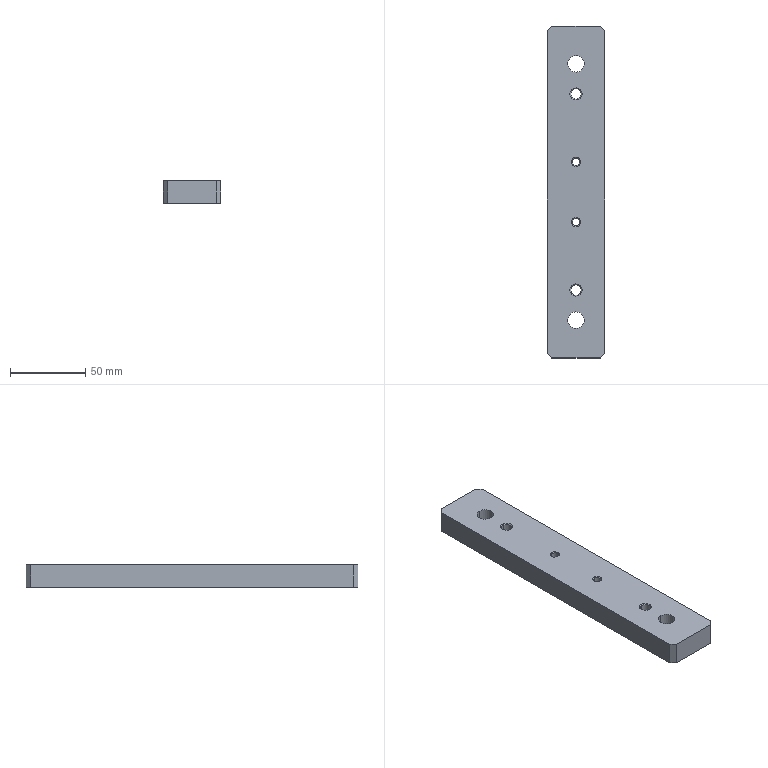Component | SolidWorks | TransitionPlate-1 | 1 solid | 30 faces | box 38 x 220 x 15 mm | volume 120587 mm3 | cylinder 12 | plane 10 | cone 8 | commonest cylinder face diameters 5 x4 6.8 x4 11 x4
build123d program:
from build123d import *

# Parameters (mm, degrees)
BOSS_EXTRUDE1_DEPTH                                  = 15
F_11_0_11_DIAMETER_HOLE1_D                           = 11
CONICAL_COUNTERSUNK_HOLE_1_FOR_M6_FLAT_H_D           = 6.8
CONICAL_COUNTERSUNK_HOLE_1_FOR_M6_FLAT_H_CSINK_D     = 8.05
CONICAL_COUNTERSUNK_HOLE_1_FOR_M6_FLAT_H_CSINK_ANGLE = 90
F_5_0_5_DIAMETER_HOLE1_D                             = 5
F_5_0_5_DIAMETER_HOLE1_CSINK_D                       = 6.05
F_5_0_5_DIAMETER_HOLE1_CSINK_ANGLE                   = 90


with BuildPart() as part:
    # Sketch1 → Boss-Extrude1 (new body)
    with BuildSketch(Plane.XY.offset(7.5)):
        Polygon((-110, 16), (-110, -16), (-107, -19), (107, -19), (110, -16), (110, 16), (107, 19), (-107, 19), align=None)
    extrude(amount=-BOSS_EXTRUDE1_DEPTH)

    # 11.0 _11_ Diameter Hole1 (through all)
    with Locations(Plane(origin=(0, 0, -7.5), x_dir=(-1, 0, 0), z_dir=(0, 0, -1))):
        with Locations((-85, 0), (85, 0)):
            Hole(F_11_0_11_DIAMETER_HOLE1_D / 2)

    # Conical Countersunk Hole 1 for M6 Flat H (through all)
    with Locations(Plane.XY.offset(7.5)):
        with Locations((65, 0), (-65, 0)):
            CounterSinkHole(CONICAL_COUNTERSUNK_HOLE_1_FOR_M6_FLAT_H_D / 2, CONICAL_COUNTERSUNK_HOLE_1_FOR_M6_FLAT_H_CSINK_D / 2, counter_sink_angle=CONICAL_COUNTERSUNK_HOLE_1_FOR_M6_FLAT_H_CSINK_ANGLE)

    # 5.0 _5_ Diameter Hole1 (through all)
    with Locations(Plane.XY.offset(7.5)):
        with Locations((20, 0), (-20, 0)):
            CounterSinkHole(F_5_0_5_DIAMETER_HOLE1_D / 2, F_5_0_5_DIAMETER_HOLE1_CSINK_D / 2, counter_sink_angle=F_5_0_5_DIAMETER_HOLE1_CSINK_ANGLE)


solid = part.part

# Placed as in the assembly
solid = solid.moved(Location((0, 0, 263.054), (0, 0, 90)))
STEP:
#1=COLOUR_RGB('',0.7922,0.8196,0.9333);
#2=FILL_AREA_STYLE_COLOUR('',#1);
#3=FILL_AREA_STYLE('',(#2));
#4=SURFACE_STYLE_FILL_AREA(#3);
#5=SURFACE_SIDE_STYLE('',(#4));
#6=SURFACE_STYLE_USAGE(.BOTH.,#5);
#7=PRESENTATION_STYLE_ASSIGNMENT((#6));
#8=CARTESIAN_POINT('',(-0.,-0.689,10.631));
#9=VERTEX_POINT('',#8);
#10=CARTESIAN_POINT('',(-0.,-0.8858,10.631));
#11=VERTEX_POINT('',#10);
#12=CARTESIAN_POINT('',(-0.,-0.7874,10.631));
#13=DIRECTION('',(-0.,0.,1.));
#14=DIRECTION('',(-0.,-1.,0.));
#15=AXIS2_PLACEMENT_3D('',#12,#13,#14);
#16=CIRCLE('',#15,0.09843);
#17=EDGE_CURVE('',#9,#11,#16,.T.);
#18=ORIENTED_EDGE('',*,*,#17,.F.);
#19=CARTESIAN_POINT('',(-0.,-0.6683,10.652));
#20=VERTEX_POINT('',#19);
#21=CARTESIAN_POINT('',(-0.,-0.6683,10.652));
#22=DIRECTION('',(0.,0.7071,0.7071));
#23=VECTOR('',#22,39.37);
#24=LINE('',#21,#23);
#25=EDGE_CURVE('',#9,#20,#24,.T.);
#26=ORIENTED_EDGE('',*,*,#25,.T.);
#27=CARTESIAN_POINT('',(-0.,-0.9065,10.652));
#28=VERTEX_POINT('',#27);
#29=CARTESIAN_POINT('',(-0.,-0.7874,10.652));
#30=DIRECTION('',(-0.,0.,1.));
#31=DIRECTION('',(-0.,-1.,0.));
#32=AXIS2_PLACEMENT_3D('',#29,#30,#31);
#33=CIRCLE('',#32,0.1191);
#34=EDGE_CURVE('',#20,#28,#33,.T.);
#35=ORIENTED_EDGE('',*,*,#34,.T.);
#36=CARTESIAN_POINT('',(-0.,-0.9065,10.652));
#37=DIRECTION('',(-0.,-0.7071,0.7071));
#38=VECTOR('',#37,39.37);
#39=LINE('',#36,#38);
#40=EDGE_CURVE('',#11,#28,#39,.T.);
#41=ORIENTED_EDGE('',*,*,#40,.F.);
#42=EDGE_LOOP('',(#18,#26,#35,#41));
#43=FACE_OUTER_BOUND('',#42,.T.);
#44=CARTESIAN_POINT('',(-0.,-0.7874,10.652));
#45=DIRECTION('',(-0.,0.,1.));
#46=DIRECTION('',(-0.,-1.,0.));
#47=AXIS2_PLACEMENT_3D('',#44,#45,#46);
#48=CONICAL_SURFACE('',#47,0.1191,0.7854);
#49=ADVANCED_FACE('',(#43),#48,.F.);
#50=CARTESIAN_POINT('',(-0.,-0.689,10.061));
#51=VERTEX_POINT('',#50);
#52=CARTESIAN_POINT('',(-0.,-0.8858,10.061));
#53=VERTEX_POINT('',#52);
#54=CARTESIAN_POINT('',(-0.,-0.7874,10.061));
#55=DIRECTION('',(-0.,0.,1.));
#56=DIRECTION('',(-0.,-1.,0.));
#57=AXIS2_PLACEMENT_3D('',#54,#55,#56);
#58=CIRCLE('',#57,0.09843);
#59=EDGE_CURVE('',#51,#53,#58,.T.);
#60=ORIENTED_EDGE('',*,*,#59,.F.);
#61=CARTESIAN_POINT('',(-0.,-0.689,10.652));
#62=DIRECTION('',(-0.,0.,1.));
#63=VECTOR('',#62,39.37);
#64=LINE('',#61,#63);
#65=EDGE_CURVE('',#51,#9,#64,.T.);
#66=ORIENTED_EDGE('',*,*,#65,.T.);
#67=ORIENTED_EDGE('',*,*,#17,.T.);
#68=CARTESIAN_POINT('',(-0.,-0.8858,10.652));
#69=DIRECTION('',(-0.,0.,1.));
#70=VECTOR('',#69,39.37);
#71=LINE('',#68,#70);
#72=EDGE_CURVE('',#53,#11,#71,.T.);
#73=ORIENTED_EDGE('',*,*,#72,.F.);
#74=EDGE_LOOP('',(#60,#66,#67,#73));
#75=FACE_OUTER_BOUND('',#74,.T.);
#76=CARTESIAN_POINT('',(-0.,-0.7874,10.652));
#77=DIRECTION('',(-0.,0.,1.));
#78=DIRECTION('',(-0.,-1.,0.));
#79=AXIS2_PLACEMENT_3D('',#76,#77,#78);
#80=CYLINDRICAL_SURFACE('',#79,0.09843);
#81=ADVANCED_FACE('',(#75),#80,.F.);
#82=CARTESIAN_POINT('',(-0.,0.8858,10.631));
#83=VERTEX_POINT('',#82);
#84=CARTESIAN_POINT('',(-0.,0.689,10.631));
#85=VERTEX_POINT('',#84);
#86=CARTESIAN_POINT('',(-0.,0.7874,10.631));
#87=DIRECTION('',(-0.,0.,1.));
#88=DIRECTION('',(-0.,-1.,0.));
#89=AXIS2_PLACEMENT_3D('',#86,#87,#88);
#90=CIRCLE('',#89,0.09843);
#91=EDGE_CURVE('',#83,#85,#90,.T.);
#92=ORIENTED_EDGE('',*,*,#91,.F.);
#93=CARTESIAN_POINT('',(-0.,0.9065,10.652));
#94=VERTEX_POINT('',#93);
#95=CARTESIAN_POINT('',(-0.,0.9065,10.652));
#96=DIRECTION('',(0.,0.7071,0.7071));
#97=VECTOR('',#96,39.37);
#98=LINE('',#95,#97);
#99=EDGE_CURVE('',#83,#94,#98,.T.);
#100=ORIENTED_EDGE('',*,*,#99,.T.);
#101=CARTESIAN_POINT('',(-0.,0.6683,10.652));
#102=VERTEX_POINT('',#101);
#103=CARTESIAN_POINT('',(-0.,0.7874,10.652));
#104=DIRECTION('',(-0.,0.,1.));
#105=DIRECTION('',(-0.,-1.,0.));
#106=AXIS2_PLACEMENT_3D('',#103,#104,#105);
#107=CIRCLE('',#106,0.1191);
#108=EDGE_CURVE('',#94,#102,#107,.T.);
#109=ORIENTED_EDGE('',*,*,#108,.T.);
#110=CARTESIAN_POINT('',(-0.,0.6683,10.652));
#111=DIRECTION('',(-0.,-0.7071,0.7071));
#112=VECTOR('',#111,39.37);
#113=LINE('',#110,#112);
#114=EDGE_CURVE('',#85,#102,#113,.T.);
#115=ORIENTED_EDGE('',*,*,#114,.F.);
#116=EDGE_LOOP('',(#92,#100,#109,#115));
#117=FACE_OUTER_BOUND('',#116,.T.);
#118=CARTESIAN_POINT('',(-0.,0.7874,10.652));
#119=DIRECTION('',(-0.,0.,1.));
#120=DIRECTION('',(-0.,-1.,0.));
#121=AXIS2_PLACEMENT_3D('',#118,#119,#120);
#122=CONICAL_SURFACE('',#121,0.1191,0.7854);
#123=ADVANCED_FACE('',(#117),#122,.F.);
#124=CARTESIAN_POINT('',(-0.,0.8858,10.061));
#125=VERTEX_POINT('',#124);
#126=CARTESIAN_POINT('',(-0.,0.689,10.061));
#127=VERTEX_POINT('',#126);
#128=CARTESIAN_POINT('',(-0.,0.7874,10.061));
#129=DIRECTION('',(-0.,0.,1.));
#130=DIRECTION('',(-0.,-1.,0.));
#131=AXIS2_PLACEMENT_3D('',#128,#129,#130);
#132=CIRCLE('',#131,0.09843);
#133=EDGE_CURVE('',#125,#127,#132,.T.);
#134=ORIENTED_EDGE('',*,*,#133,.F.);
#135=CARTESIAN_POINT('',(-0.,0.8858,10.652));
#136=DIRECTION('',(-0.,0.,1.));
#137=VECTOR('',#136,39.37);
#138=LINE('',#135,#137);
#139=EDGE_CURVE('',#125,#83,#138,.T.);
#140=ORIENTED_EDGE('',*,*,#139,.T.);
#141=ORIENTED_EDGE('',*,*,#91,.T.);
#142=CARTESIAN_POINT('',(-0.,0.689,10.652));
#143=DIRECTION('',(-0.,0.,1.));
#144=VECTOR('',#143,39.37);
#145=LINE('',#142,#144);
#146=EDGE_CURVE('',#127,#85,#145,.T.);
#147=ORIENTED_EDGE('',*,*,#146,.F.);
#148=EDGE_LOOP('',(#134,#140,#141,#147));
#149=FACE_OUTER_BOUND('',#148,.T.);
#150=CARTESIAN_POINT('',(-0.,0.7874,10.652));
#151=DIRECTION('',(-0.,0.,1.));
#152=DIRECTION('',(-0.,-1.,0.));
#153=AXIS2_PLACEMENT_3D('',#150,#151,#152);
#154=CYLINDRICAL_SURFACE('',#153,0.09843);
#155=ADVANCED_FACE('',(#149),#154,.F.);
#156=CARTESIAN_POINT('',(-0.,-2.425,10.627));
#157=VERTEX_POINT('',#156);
#158=CARTESIAN_POINT('',(-0.,-2.693,10.627));
#159=VERTEX_POINT('',#158);
#160=CARTESIAN_POINT('',(-0.,-2.559,10.627));
#161=DIRECTION('',(-0.,0.,1.));
#162=DIRECTION('',(-0.,-1.,0.));
#163=AXIS2_PLACEMENT_3D('',#160,#161,#162);
#164=CIRCLE('',#163,0.1339);
#165=EDGE_CURVE('',#157,#159,#164,.T.);
#166=ORIENTED_EDGE('',*,*,#165,.F.);
#167=CARTESIAN_POINT('',(-0.,-2.401,10.652));
#168=VERTEX_POINT('',#167);
#169=CARTESIAN_POINT('',(-0.,-2.401,10.652));
#170=DIRECTION('',(0.,0.7071,0.7071));
#171=VECTOR('',#170,39.37);
#172=LINE('',#169,#171);
#173=EDGE_CURVE('',#157,#168,#172,.T.);
#174=ORIENTED_EDGE('',*,*,#173,.T.);
#175=CARTESIAN_POINT('',(-0.,-2.718,10.652));
#176=VERTEX_POINT('',#175);
#177=CARTESIAN_POINT('',(-0.,-2.559,10.652));
#178=DIRECTION('',(-0.,0.,1.));
#179=DIRECTION('',(-0.,-1.,0.));
#180=AXIS2_PLACEMENT_3D('',#177,#178,#179);
#181=CIRCLE('',#180,0.1585);
#182=EDGE_CURVE('',#168,#176,#181,.T.);
#183=ORIENTED_EDGE('',*,*,#182,.T.);
#184=CARTESIAN_POINT('',(-0.,-2.718,10.652));
#185=DIRECTION('',(-0.,-0.7071,0.7071));
#186=VECTOR('',#185,39.37);
#187=LINE('',#184,#186);
#188=EDGE_CURVE('',#159,#176,#187,.T.);
#189=ORIENTED_EDGE('',*,*,#188,.F.);
#190=EDGE_LOOP('',(#166,#174,#183,#189));
#191=FACE_OUTER_BOUND('',#190,.T.);
#192=CARTESIAN_POINT('',(-0.,-2.559,10.652));
#193=DIRECTION('',(-0.,0.,1.));
#194=DIRECTION('',(-0.,-1.,0.));
#195=AXIS2_PLACEMENT_3D('',#192,#193,#194);
#196=CONICAL_SURFACE('',#195,0.1585,0.7854);
#197=ADVANCED_FACE('',(#191),#196,.F.);
#198=CARTESIAN_POINT('',(-0.,-2.425,10.061));
#199=VERTEX_POINT('',#198);
#200=CARTESIAN_POINT('',(-0.,-2.693,10.061));
#201=VERTEX_POINT('',#200);
#202=CARTESIAN_POINT('',(-0.,-2.559,10.061));
#203=DIRECTION('',(-0.,0.,1.));
#204=DIRECTION('',(-0.,-1.,0.));
#205=AXIS2_PLACEMENT_3D('',#202,#203,#204);
#206=CIRCLE('',#205,0.1339);
#207=EDGE_CURVE('',#199,#201,#206,.T.);
#208=ORIENTED_EDGE('',*,*,#207,.F.);
#209=CARTESIAN_POINT('',(-0.,-2.425,10.652));
#210=DIRECTION('',(-0.,0.,1.));
#211=VECTOR('',#210,39.37);
#212=LINE('',#209,#211);
#213=EDGE_CURVE('',#199,#157,#212,.T.);
#214=ORIENTED_EDGE('',*,*,#213,.T.);
#215=ORIENTED_EDGE('',*,*,#165,.T.);
#216=CARTESIAN_POINT('',(-0.,-2.693,10.652));
#217=DIRECTION('',(-0.,0.,1.));
#218=VECTOR('',#217,39.37);
#219=LINE('',#216,#218);
#220=EDGE_CURVE('',#201,#159,#219,.T.);
#221=ORIENTED_EDGE('',*,*,#220,.F.);
#222=EDGE_LOOP('',(#208,#214,#215,#221));
#223=FACE_OUTER_BOUND('',#222,.T.);
#224=CARTESIAN_POINT('',(-0.,-2.559,10.652));
#225=DIRECTION('',(-0.,0.,1.));
#226=DIRECTION('',(-0.,-1.,0.));
#227=AXIS2_PLACEMENT_3D('',#224,#225,#226);
#228=CYLINDRICAL_SURFACE('',#227,0.1339);
#229=ADVANCED_FACE('',(#223),#228,.F.);
#230=CARTESIAN_POINT('',(-0.,2.693,10.627));
#231=VERTEX_POINT('',#230);
#232=CARTESIAN_POINT('',(-0.,2.425,10.627));
#233=VERTEX_POINT('',#232);
#234=CARTESIAN_POINT('',(-0.,2.559,10.627));
#235=DIRECTION('',(-0.,0.,1.));
#236=DIRECTION('',(-0.,-1.,0.));
#237=AXIS2_PLACEMENT_3D('',#234,#235,#236);
#238=CIRCLE('',#237,0.1339);
#239=EDGE_CURVE('',#231,#233,#238,.T.);
#240=ORIENTED_EDGE('',*,*,#239,.F.);
#241=CARTESIAN_POINT('',(-0.,2.718,10.652));
#242=VERTEX_POINT('',#241);
#243=CARTESIAN_POINT('',(-0.,2.718,10.652));
#244=DIRECTION('',(0.,0.7071,0.7071));
#245=VECTOR('',#244,39.37);
#246=LINE('',#243,#245);
#247=EDGE_CURVE('',#231,#242,#246,.T.);
#248=ORIENTED_EDGE('',*,*,#247,.T.);
#249=CARTESIAN_POINT('',(-0.,2.401,10.652));
#250=VERTEX_POINT('',#249);
#251=CARTESIAN_POINT('',(-0.,2.559,10.652));
#252=DIRECTION('',(-0.,0.,1.));
#253=DIRECTION('',(-0.,-1.,0.));
#254=AXIS2_PLACEMENT_3D('',#251,#252,#253);
#255=CIRCLE('',#254,0.1585);
#256=EDGE_CURVE('',#242,#250,#255,.T.);
#257=ORIENTED_EDGE('',*,*,#256,.T.);
#258=CARTESIAN_POINT('',(-0.,2.401,10.652));
#259=DIRECTION('',(-0.,-0.7071,0.7071));
#260=VECTOR('',#259,39.37);
#261=LINE('',#258,#260);
#262=EDGE_CURVE('',#233,#250,#261,.T.);
#263=ORIENTED_EDGE('',*,*,#262,.F.);
#264=EDGE_LOOP('',(#240,#248,#257,#263));
#265=FACE_OUTER_BOUND('',#264,.T.);
#266=CARTESIAN_POINT('',(-0.,2.559,10.652));
#267=DIRECTION('',(-0.,0.,1.));
#268=DIRECTION('',(-0.,-1.,0.));
#269=AXIS2_PLACEMENT_3D('',#266,#267,#268);
#270=CONICAL_SURFACE('',#269,0.1585,0.7854);
#271=ADVANCED_FACE('',(#265),#270,.F.);
#272=CARTESIAN_POINT('',(-0.,2.693,10.061));
#273=VERTEX_POINT('',#272);
#274=CARTESIAN_POINT('',(-0.,2.425,10.061));
#275=VERTEX_POINT('',#274);
#276=CARTESIAN_POINT('',(-0.,2.559,10.061));
#277=DIRECTION('',(-0.,0.,1.));
#278=DIRECTION('',(-0.,-1.,0.));
#279=AXIS2_PLACEMENT_3D('',#276,#277,#278);
#280=CIRCLE('',#279,0.1339);
#281=EDGE_CURVE('',#273,#275,#280,.T.);
#282=ORIENTED_EDGE('',*,*,#281,.F.);
#283=CARTESIAN_POINT('',(-0.,2.693,10.652));
#284=DIRECTION('',(-0.,0.,1.));
#285=VECTOR('',#284,39.37);
#286=LINE('',#283,#285);
#287=EDGE_CURVE('',#273,#231,#286,.T.);
#288=ORIENTED_EDGE('',*,*,#287,.T.);
#289=ORIENTED_EDGE('',*,*,#239,.T.);
#290=CARTESIAN_POINT('',(-0.,2.425,10.652));
#291=DIRECTION('',(-0.,0.,1.));
#292=VECTOR('',#291,39.37);
#293=LINE('',#290,#292);
#294=EDGE_CURVE('',#275,#233,#293,.T.);
#295=ORIENTED_EDGE('',*,*,#294,.F.);
#296=EDGE_LOOP('',(#282,#288,#289,#295));
#297=FACE_OUTER_BOUND('',#296,.T.);
#298=CARTESIAN_POINT('',(-0.,2.559,10.652));
#299=DIRECTION('',(-0.,0.,1.));
#300=DIRECTION('',(-0.,-1.,0.));
#301=AXIS2_PLACEMENT_3D('',#298,#299,#300);
#302=CYLINDRICAL_SURFACE('',#301,0.1339);
#303=ADVANCED_FACE('',(#297),#302,.F.);
#304=CARTESIAN_POINT('',(-0.,-3.563,10.652));
#305=VERTEX_POINT('',#304);
#306=CARTESIAN_POINT('',(-0.,-3.13,10.652));
#307=VERTEX_POINT('',#306);
#308=CARTESIAN_POINT('',(-0.,-3.346,10.652));
#309=DIRECTION('',(0.,-0.,-1.));
#310=DIRECTION('',(0.,1.,0.));
#311=AXIS2_PLACEMENT_3D('',#308,#309,#310);
#312=CIRCLE('',#311,0.2165);
#313=EDGE_CURVE('',#305,#307,#312,.T.);
#314=ORIENTED_EDGE('',*,*,#313,.F.);
#315=CARTESIAN_POINT('',(-0.,-3.563,10.061));
#316=VERTEX_POINT('',#315);
#317=CARTESIAN_POINT('',(-0.,-3.563,10.061));
#318=DIRECTION('',(0.,-0.,-1.));
#319=VECTOR('',#318,39.37);
#320=LINE('',#317,#319);
#321=EDGE_CURVE('',#305,#316,#320,.T.);
#322=ORIENTED_EDGE('',*,*,#321,.T.);
#323=CARTESIAN_POINT('',(-0.,-3.13,10.061));
#324=VERTEX_POINT('',#323);
#325=CARTESIAN_POINT('',(-0.,-3.346,10.061));
#326=DIRECTION('',(0.,-0.,-1.));
#327=DIRECTION('',(0.,1.,0.));
#328=AXIS2_PLACEMENT_3D('',#325,#326,#327);
#329=CIRCLE('',#328,0.2165);
#330=EDGE_CURVE('',#316,#324,#329,.T.);
#331=ORIENTED_EDGE('',*,*,#330,.T.);
#332=CARTESIAN_POINT('',(-0.,-3.13,10.061));
#333=DIRECTION('',(0.,-0.,-1.));
#334=VECTOR('',#333,39.37);
#335=LINE('',#332,#334);
#336=EDGE_CURVE('',#307,#324,#335,.T.);
#337=ORIENTED_EDGE('',*,*,#336,.F.);
#338=EDGE_LOOP('',(#314,#322,#331,#337));
#339=FACE_OUTER_BOUND('',#338,.T.);
#340=CARTESIAN_POINT('',(-0.,-3.346,10.061));
#341=DIRECTION('',(0.,-0.,-1.));
#342=DIRECTION('',(0.,1.,0.));
#343=AXIS2_PLACEMENT_3D('',#340,#341,#342);
#344=CYLINDRICAL_SURFACE('',#343,0.2165);
#345=ADVANCED_FACE('',(#339),#344,.F.);
#346=CARTESIAN_POINT('',(-0.,3.13,10.652));
#347=VERTEX_POINT('',#346);
#348=CARTESIAN_POINT('',(-0.,3.563,10.652));
#349=VERTEX_POINT('',#348);
#350=CARTESIAN_POINT('',(-0.,3.346,10.652));
#351=DIRECTION('',(0.,-0.,-1.));
#352=DIRECTION('',(0.,1.,0.));
#353=AXIS2_PLACEMENT_3D('',#350,#351,#352);
#354=CIRCLE('',#353,0.2165);
#355=EDGE_CURVE('',#347,#349,#354,.T.);
#356=ORIENTED_EDGE('',*,*,#355,.F.);
#357=CARTESIAN_POINT('',(-0.,3.13,10.061));
#358=VERTEX_POINT('',#357);
#359=CARTESIAN_POINT('',(-0.,3.13,10.061));
#360=DIRECTION('',(0.,-0.,-1.));
#361=VECTOR('',#360,39.37);
#362=LINE('',#359,#361);
#363=EDGE_CURVE('',#347,#358,#362,.T.);
#364=ORIENTED_EDGE('',*,*,#363,.T.);
#365=CARTESIAN_POINT('',(-0.,3.563,10.061));
#366=VERTEX_POINT('',#365);
#367=CARTESIAN_POINT('',(-0.,3.346,10.061));
#368=DIRECTION('',(0.,-0.,-1.));
#369=DIRECTION('',(0.,1.,0.));
#370=AXIS2_PLACEMENT_3D('',#367,#368,#369);
#371=CIRCLE('',#370,0.2165);
#372=EDGE_CURVE('',#358,#366,#371,.T.);
#373=ORIENTED_EDGE('',*,*,#372,.T.);
#374=CARTESIAN_POINT('',(-0.,3.563,10.061));
#375=DIRECTION('',(0.,-0.,-1.));
#376=VECTOR('',#375,39.37);
#377=LINE('',#374,#376);
#378=EDGE_CURVE('',#349,#366,#377,.T.);
#379=ORIENTED_EDGE('',*,*,#378,.F.);
#380=EDGE_LOOP('',(#356,#364,#373,#379));
#381=FACE_OUTER_BOUND('',#380,.T.);
#382=CARTESIAN_POINT('',(-0.,3.346,10.061));
#383=DIRECTION('',(0.,-0.,-1.));
#384=DIRECTION('',(0.,1.,0.));
#385=AXIS2_PLACEMENT_3D('',#382,#383,#384);
#386=CYLINDRICAL_SURFACE('',#385,0.2165);
#387=ADVANCED_FACE('',(#381),#386,.F.);
#388=CARTESIAN_POINT('',(0.748,4.213,10.652));
#389=VERTEX_POINT('',#388);
#390=CARTESIAN_POINT('',(0.6299,4.331,10.652));
#391=VERTEX_POINT('',#390);
#392=CARTESIAN_POINT('',(0.748,4.213,10.652));
#393=DIRECTION('',(-0.7071,0.7071,-0.));
#394=VECTOR('',#393,39.37);
#395=LINE('',#392,#394);
#396=EDGE_CURVE('',#389,#391,#395,.T.);
#397=ORIENTED_EDGE('',*,*,#396,.F.);
#398=CARTESIAN_POINT('',(0.748,4.213,10.061));
#399=VERTEX_POINT('',#398);
#400=CARTESIAN_POINT('',(0.748,4.213,10.061));
#401=DIRECTION('',(-0.,0.,1.));
#402=VECTOR('',#401,39.37);
#403=LINE('',#400,#402);
#404=EDGE_CURVE('',#399,#389,#403,.T.);
#405=ORIENTED_EDGE('',*,*,#404,.F.);
#406=CARTESIAN_POINT('',(0.6299,4.331,10.061));
#407=VERTEX_POINT('',#406);
#408=CARTESIAN_POINT('',(0.748,4.213,10.061));
#409=DIRECTION('',(-0.7071,0.7071,-0.));
#410=VECTOR('',#409,39.37);
#411=LINE('',#408,#410);
#412=EDGE_CURVE('',#399,#407,#411,.T.);
#413=ORIENTED_EDGE('',*,*,#412,.T.);
#414=CARTESIAN_POINT('',(0.6299,4.331,10.061));
#415=DIRECTION('',(-0.,0.,1.));
#416=VECTOR('',#415,39.37);
#417=LINE('',#414,#416);
#418=EDGE_CURVE('',#407,#391,#417,.T.);
#419=ORIENTED_EDGE('',*,*,#418,.T.);
#420=EDGE_LOOP('',(#397,#405,#413,#419));
#421=FACE_OUTER_BOUND('',#420,.T.);
#422=CARTESIAN_POINT('',(0.748,4.213,10.061));
#423=DIRECTION('',(0.7071,0.7071,0.));
#424=DIRECTION('',(-0.7071,0.7071,-0.));
#425=AXIS2_PLACEMENT_3D('',#422,#423,#424);
#426=PLANE('',#425);
#427=ADVANCED_FACE('',(#421),#426,.T.);
#428=CARTESIAN_POINT('',(0.748,-4.213,10.652));
#429=VERTEX_POINT('',#428);
#430=CARTESIAN_POINT('',(0.748,-4.213,10.652));
#431=DIRECTION('',(0.,1.,-0.));
#432=VECTOR('',#431,39.37);
#433=LINE('',#430,#432);
#434=EDGE_CURVE('',#429,#389,#433,.T.);
#435=ORIENTED_EDGE('',*,*,#434,.F.);
#436=CARTESIAN_POINT('',(0.748,-4.213,10.061));
#437=VERTEX_POINT('',#436);
#438=CARTESIAN_POINT('',(0.748,-4.213,10.061));
#439=DIRECTION('',(-0.,0.,1.));
#440=VECTOR('',#439,39.37);
#441=LINE('',#438,#440);
#442=EDGE_CURVE('',#437,#429,#441,.T.);
#443=ORIENTED_EDGE('',*,*,#442,.F.);
#444=CARTESIAN_POINT('',(0.748,-4.213,10.061));
#445=DIRECTION('',(0.,1.,-0.));
#446=VECTOR('',#445,39.37);
#447=LINE('',#444,#446);
#448=EDGE_CURVE('',#437,#399,#447,.T.);
#449=ORIENTED_EDGE('',*,*,#448,.T.);
#450=ORIENTED_EDGE('',*,*,#404,.T.);
#451=EDGE_LOOP('',(#435,#443,#449,#450));
#452=FACE_OUTER_BOUND('',#451,.T.);
#453=CARTESIAN_POINT('',(0.748,-4.213,10.061));
#454=DIRECTION('',(1.,-0.,0.));
#455=DIRECTION('',(-0.,0.,1.));
#456=AXIS2_PLACEMENT_3D('',#453,#454,#455);
#457=PLANE('',#456);
#458=ADVANCED_FACE('',(#452),#457,.T.);
#459=CARTESIAN_POINT('',(0.6299,-4.331,10.652));
#460=VERTEX_POINT('',#459);
#461=CARTESIAN_POINT('',(0.6299,-4.331,10.652));
#462=DIRECTION('',(0.7071,0.7071,0.));
#463=VECTOR('',#462,39.37);
#464=LINE('',#461,#463);
#465=EDGE_CURVE('',#460,#429,#464,.T.);
#466=ORIENTED_EDGE('',*,*,#465,.F.);
#467=CARTESIAN_POINT('',(0.6299,-4.331,10.061));
#468=VERTEX_POINT('',#467);
#469=CARTESIAN_POINT('',(0.6299,-4.331,10.061));
#470=DIRECTION('',(-0.,0.,1.));
#471=VECTOR('',#470,39.37);
#472=LINE('',#469,#471);
#473=EDGE_CURVE('',#468,#460,#472,.T.);
#474=ORIENTED_EDGE('',*,*,#473,.F.);
#475=CARTESIAN_POINT('',(0.6299,-4.331,10.061));
#476=DIRECTION('',(0.7071,0.7071,0.));
#477=VECTOR('',#476,39.37);
#478=LINE('',#475,#477);
#479=EDGE_CURVE('',#468,#437,#478,.T.);
#480=ORIENTED_EDGE('',*,*,#479,.T.);
#481=ORIENTED_EDGE('',*,*,#442,.T.);
#482=EDGE_LOOP('',(#466,#474,#480,#481));
#483=FACE_OUTER_BOUND('',#482,.T.);
#484=CARTESIAN_POINT('',(0.6299,-4.331,10.061));
#485=DIRECTION('',(0.7071,-0.7071,0.));
#486=DIRECTION('',(0.7071,0.7071,0.));
#487=AXIS2_PLACEMENT_3D('',#484,#485,#486);
#488=PLANE('',#487);
#489=ADVANCED_FACE('',(#483),#488,.T.);
#490=CARTESIAN_POINT('',(-0.6299,-4.331,10.652));
#491=VERTEX_POINT('',#490);
#492=CARTESIAN_POINT('',(-0.6299,-4.331,10.652));
#493=DIRECTION('',(1.,-0.,0.));
#494=VECTOR('',#493,39.37);
#495=LINE('',#492,#494);
#496=EDGE_CURVE('',#491,#460,#495,.T.);
#497=ORIENTED_EDGE('',*,*,#496,.F.);
#498=CARTESIAN_POINT('',(-0.6299,-4.331,10.061));
#499=VERTEX_POINT('',#498);
#500=CARTESIAN_POINT('',(-0.6299,-4.331,10.061));
#501=DIRECTION('',(-0.,0.,1.));
#502=VECTOR('',#501,39.37);
#503=LINE('',#500,#502);
#504=EDGE_CURVE('',#499,#491,#503,.T.);
#505=ORIENTED_EDGE('',*,*,#504,.F.);
#506=CARTESIAN_POINT('',(-0.6299,-4.331,10.061));
#507=DIRECTION('',(1.,-0.,0.));
#508=VECTOR('',#507,39.37);
#509=LINE('',#506,#508);
#510=EDGE_CURVE('',#499,#468,#509,.T.);
#511=ORIENTED_EDGE('',*,*,#510,.T.);
#512=ORIENTED_EDGE('',*,*,#473,.T.);
#513=EDGE_LOOP('',(#497,#505,#511,#512));
#514=FACE_OUTER_BOUND('',#513,.T.);
#515=CARTESIAN_POINT('',(-0.6299,-4.331,10.061));
#516=DIRECTION('',(-0.,-1.,0.));
#517=DIRECTION('',(0.,-0.,-1.));
#518=AXIS2_PLACEMENT_3D('',#515,#516,#517);
#519=PLANE('',#518);
#520=ADVANCED_FACE('',(#514),#519,.T.);
#521=CARTESIAN_POINT('',(-0.748,-4.213,10.652));
#522=VERTEX_POINT('',#521);
#523=CARTESIAN_POINT('',(-0.748,-4.213,10.652));
#524=DIRECTION('',(0.7071,-0.7071,0.));
#525=VECTOR('',#524,39.37);
#526=LINE('',#523,#525);
#527=EDGE_CURVE('',#522,#491,#526,.T.);
#528=ORIENTED_EDGE('',*,*,#527,.F.);
#529=CARTESIAN_POINT('',(-0.748,-4.213,10.061));
#530=VERTEX_POINT('',#529);
#531=CARTESIAN_POINT('',(-0.748,-4.213,10.061));
#532=DIRECTION('',(-0.,0.,1.));
#533=VECTOR('',#532,39.37);
#534=LINE('',#531,#533);
#535=EDGE_CURVE('',#530,#522,#534,.T.);
#536=ORIENTED_EDGE('',*,*,#535,.F.);
#537=CARTESIAN_POINT('',(-0.748,-4.213,10.061));
#538=DIRECTION('',(0.7071,-0.7071,0.));
#539=VECTOR('',#538,39.37);
#540=LINE('',#537,#539);
#541=EDGE_CURVE('',#530,#499,#540,.T.);
#542=ORIENTED_EDGE('',*,*,#541,.T.);
#543=ORIENTED_EDGE('',*,*,#504,.T.);
#544=EDGE_LOOP('',(#528,#536,#542,#543));
#545=FACE_OUTER_BOUND('',#544,.T.);
#546=CARTESIAN_POINT('',(-0.748,-4.213,10.061));
#547=DIRECTION('',(-0.7071,-0.7071,-0.));
#548=DIRECTION('',(0.7071,-0.7071,0.));
#549=AXIS2_PLACEMENT_3D('',#546,#547,#548);
#550=PLANE('',#549);
#551=ADVANCED_FACE('',(#545),#550,.T.);
#552=CARTESIAN_POINT('',(-0.748,4.213,10.652));
#553=VERTEX_POINT('',#552);
#554=CARTESIAN_POINT('',(-0.748,4.213,10.652));
#555=DIRECTION('',(-0.,-1.,0.));
#556=VECTOR('',#555,39.37);
#557=LINE('',#554,#556);
#558=EDGE_CURVE('',#553,#522,#557,.T.);
#559=ORIENTED_EDGE('',*,*,#558,.F.);
#560=CARTESIAN_POINT('',(-0.748,4.213,10.061));
#561=VERTEX_POINT('',#560);
#562=CARTESIAN_POINT('',(-0.748,4.213,10.061));
#563=DIRECTION('',(-0.,0.,1.));
#564=VECTOR('',#563,39.37);
#565=LINE('',#562,#564);
#566=EDGE_CURVE('',#561,#553,#565,.T.);
#567=ORIENTED_EDGE('',*,*,#566,.F.);
#568=CARTESIAN_POINT('',(-0.748,4.213,10.061));
#569=DIRECTION('',(-0.,-1.,0.));
#570=VECTOR('',#569,39.37);
#571=LINE('',#568,#570);
#572=EDGE_CURVE('',#561,#530,#571,.T.);
#573=ORIENTED_EDGE('',*,*,#572,.T.);
#574=ORIENTED_EDGE('',*,*,#535,.T.);
#575=EDGE_LOOP('',(#559,#567,#573,#574));
#576=FACE_OUTER_BOUND('',#575,.T.);
#577=CARTESIAN_POINT('',(-0.748,4.213,10.061));
#578=DIRECTION('',(-1.,0.,-0.));
#579=DIRECTION('',(0.,-0.,-1.));
#580=AXIS2_PLACEMENT_3D('',#577,#578,#579);
#581=PLANE('',#580);
#582=ADVANCED_FACE('',(#576),#581,.T.);
#583=CARTESIAN_POINT('',(-0.6299,4.331,10.652));
#584=VERTEX_POINT('',#583);
#585=CARTESIAN_POINT('',(-0.6299,4.331,10.652));
#586=DIRECTION('',(-0.7071,-0.7071,-0.));
#587=VECTOR('',#586,39.37);
#588=LINE('',#585,#587);
#589=EDGE_CURVE('',#584,#553,#588,.T.);
#590=ORIENTED_EDGE('',*,*,#589,.F.);
#591=CARTESIAN_POINT('',(-0.6299,4.331,10.061));
#592=VERTEX_POINT('',#591);
#593=CARTESIAN_POINT('',(-0.6299,4.331,10.061));
#594=DIRECTION('',(-0.,0.,1.));
#595=VECTOR('',#594,39.37);
#596=LINE('',#593,#595);
#597=EDGE_CURVE('',#592,#584,#596,.T.);
#598=ORIENTED_EDGE('',*,*,#597,.F.);
#599=CARTESIAN_POINT('',(-0.6299,4.331,10.061));
#600=DIRECTION('',(-0.7071,-0.7071,-0.));
#601=VECTOR('',#600,39.37);
#602=LINE('',#599,#601);
#603=EDGE_CURVE('',#592,#561,#602,.T.);
#604=ORIENTED_EDGE('',*,*,#603,.T.);
#605=ORIENTED_EDGE('',*,*,#566,.T.);
#606=EDGE_LOOP('',(#590,#598,#604,#605));
#607=FACE_OUTER_BOUND('',#606,.T.);
#608=CARTESIAN_POINT('',(-0.6299,4.331,10.061));
#609=DIRECTION('',(-0.7071,0.7071,-0.));
#610=DIRECTION('',(-0.7071,-0.7071,-0.));
#611=AXIS2_PLACEMENT_3D('',#608,#609,#610);
#612=PLANE('',#611);
#613=ADVANCED_FACE('',(#607),#612,.T.);
#614=CARTESIAN_POINT('',(0.6299,4.331,10.652));
#615=DIRECTION('',(-1.,0.,-0.));
#616=VECTOR('',#615,39.37);
#617=LINE('',#614,#616);
#618=EDGE_CURVE('',#391,#584,#617,.T.);
#619=ORIENTED_EDGE('',*,*,#618,.F.);
#620=ORIENTED_EDGE('',*,*,#418,.F.);
#621=CARTESIAN_POINT('',(0.6299,4.331,10.061));
#622=DIRECTION('',(-1.,0.,-0.));
#623=VECTOR('',#622,39.37);
#624=LINE('',#621,#623);
#625=EDGE_CURVE('',#407,#592,#624,.T.);
#626=ORIENTED_EDGE('',*,*,#625,.T.);
#627=ORIENTED_EDGE('',*,*,#597,.T.);
#628=EDGE_LOOP('',(#619,#620,#626,#627));
#629=FACE_OUTER_BOUND('',#628,.T.);
#630=CARTESIAN_POINT('',(0.6299,4.331,10.061));
#631=DIRECTION('',(0.,1.,-0.));
#632=DIRECTION('',(-1.,0.,-0.));
#633=AXIS2_PLACEMENT_3D('',#630,#631,#632);
#634=PLANE('',#633);
#635=ADVANCED_FACE('',(#629),#634,.T.);
#636=CARTESIAN_POINT('',(-0.,-0.7874,10.061));
#637=DIRECTION('',(-0.,0.,1.));
#638=DIRECTION('',(-0.,-1.,0.));
#639=AXIS2_PLACEMENT_3D('',#636,#637,#638);
#640=CIRCLE('',#639,0.09843);
#641=EDGE_CURVE('',#53,#51,#640,.T.);
#642=ORIENTED_EDGE('',*,*,#641,.T.);
#643=ORIENTED_EDGE('',*,*,#59,.T.);
#644=EDGE_LOOP('',(#642,#643));
#645=FACE_BOUND('',#644,.T.);
#646=CARTESIAN_POINT('',(-0.,0.7874,10.061));
#647=DIRECTION('',(-0.,0.,1.));
#648=DIRECTION('',(-0.,-1.,0.));
#649=AXIS2_PLACEMENT_3D('',#646,#647,#648);
#650=CIRCLE('',#649,0.09843);
#651=EDGE_CURVE('',#127,#125,#650,.T.);
#652=ORIENTED_EDGE('',*,*,#651,.T.);
#653=ORIENTED_EDGE('',*,*,#133,.T.);
#654=EDGE_LOOP('',(#652,#653));
#655=FACE_BOUND('',#654,.T.);
#656=CARTESIAN_POINT('',(-0.,-2.559,10.061));
#657=DIRECTION('',(-0.,0.,1.));
#658=DIRECTION('',(-0.,-1.,0.));
#659=AXIS2_PLACEMENT_3D('',#656,#657,#658);
#660=CIRCLE('',#659,0.1339);
#661=EDGE_CURVE('',#201,#199,#660,.T.);
#662=ORIENTED_EDGE('',*,*,#661,.T.);
#663=ORIENTED_EDGE('',*,*,#207,.T.);
#664=EDGE_LOOP('',(#662,#663));
#665=FACE_BOUND('',#664,.T.);
#666=CARTESIAN_POINT('',(-0.,2.559,10.061));
#667=DIRECTION('',(-0.,0.,1.));
#668=DIRECTION('',(-0.,-1.,0.));
#669=AXIS2_PLACEMENT_3D('',#666,#667,#668);
#670=CIRCLE('',#669,0.1339);
#671=EDGE_CURVE('',#275,#273,#670,.T.);
#672=ORIENTED_EDGE('',*,*,#671,.T.);
#673=ORIENTED_EDGE('',*,*,#281,.T.);
#674=EDGE_LOOP('',(#672,#673));
#675=FACE_BOUND('',#674,.T.);
#676=CARTESIAN_POINT('',(-0.,-3.346,10.061));
#677=DIRECTION('',(0.,-0.,-1.));
#678=DIRECTION('',(0.,1.,0.));
#679=AXIS2_PLACEMENT_3D('',#676,#677,#678);
#680=CIRCLE('',#679,0.2165);
#681=EDGE_CURVE('',#324,#316,#680,.T.);
#682=ORIENTED_EDGE('',*,*,#681,.F.);
#683=ORIENTED_EDGE('',*,*,#330,.F.);
#684=EDGE_LOOP('',(#682,#683));
#685=FACE_BOUND('',#684,.T.);
#686=CARTESIAN_POINT('',(-0.,3.346,10.061));
#687=DIRECTION('',(0.,-0.,-1.));
#688=DIRECTION('',(0.,1.,0.));
#689=AXIS2_PLACEMENT_3D('',#686,#687,#688);
#690=CIRCLE('',#689,0.2165);
#691=EDGE_CURVE('',#366,#358,#690,.T.);
#692=ORIENTED_EDGE('',*,*,#691,.F.);
#693=ORIENTED_EDGE('',*,*,#372,.F.);
#694=EDGE_LOOP('',(#692,#693));
#695=FACE_BOUND('',#694,.T.);
#696=ORIENTED_EDGE('',*,*,#412,.F.);
#697=ORIENTED_EDGE('',*,*,#448,.F.);
#698=ORIENTED_EDGE('',*,*,#479,.F.);
#699=ORIENTED_EDGE('',*,*,#510,.F.);
#700=ORIENTED_EDGE('',*,*,#541,.F.);
#701=ORIENTED_EDGE('',*,*,#572,.F.);
#702=ORIENTED_EDGE('',*,*,#603,.F.);
#703=ORIENTED_EDGE('',*,*,#625,.F.);
#704=EDGE_LOOP('',(#696,#697,#698,#699,#700,#701,#702,#703));
#705=FACE_OUTER_BOUND('',#704,.T.);
#706=CARTESIAN_POINT('',(-0.,-0.,10.061));
#707=DIRECTION('',(-0.,0.,1.));
#708=DIRECTION('',(-0.,-1.,0.));
#709=AXIS2_PLACEMENT_3D('',#706,#707,#708);
#710=PLANE('',#709);
#711=ADVANCED_FACE('',(#645,#655,#665,#675,#685,#695,#705),#710,.F.);
#712=CARTESIAN_POINT('',(-0.,-0.7874,10.652));
#713=DIRECTION('',(-0.,0.,1.));
#714=DIRECTION('',(-0.,-1.,0.));
#715=AXIS2_PLACEMENT_3D('',#712,#713,#714);
#716=CIRCLE('',#715,0.1191);
#717=EDGE_CURVE('',#28,#20,#716,.T.);
#718=ORIENTED_EDGE('',*,*,#717,.F.);
#719=ORIENTED_EDGE('',*,*,#34,.F.);
#720=EDGE_LOOP('',(#718,#719));
#721=FACE_BOUND('',#720,.T.);
#722=CARTESIAN_POINT('',(-0.,0.7874,10.652));
#723=DIRECTION('',(-0.,0.,1.));
#724=DIRECTION('',(-0.,-1.,0.));
#725=AXIS2_PLACEMENT_3D('',#722,#723,#724);
#726=CIRCLE('',#725,0.1191);
#727=EDGE_CURVE('',#102,#94,#726,.T.);
#728=ORIENTED_EDGE('',*,*,#727,.F.);
#729=ORIENTED_EDGE('',*,*,#108,.F.);
#730=EDGE_LOOP('',(#728,#729));
#731=FACE_BOUND('',#730,.T.);
#732=CARTESIAN_POINT('',(-0.,-2.559,10.652));
#733=DIRECTION('',(-0.,0.,1.));
#734=DIRECTION('',(-0.,-1.,0.));
#735=AXIS2_PLACEMENT_3D('',#732,#733,#734);
#736=CIRCLE('',#735,0.1585);
#737=EDGE_CURVE('',#176,#168,#736,.T.);
#738=ORIENTED_EDGE('',*,*,#737,.F.);
#739=ORIENTED_EDGE('',*,*,#182,.F.);
#740=EDGE_LOOP('',(#738,#739));
#741=FACE_BOUND('',#740,.T.);
#742=CARTESIAN_POINT('',(-0.,2.559,10.652));
#743=DIRECTION('',(-0.,0.,1.));
#744=DIRECTION('',(-0.,-1.,0.));
#745=AXIS2_PLACEMENT_3D('',#742,#743,#744);
#746=CIRCLE('',#745,0.1585);
#747=EDGE_CURVE('',#250,#242,#746,.T.);
#748=ORIENTED_EDGE('',*,*,#747,.F.);
#749=ORIENTED_EDGE('',*,*,#256,.F.);
#750=EDGE_LOOP('',(#748,#749));
#751=FACE_BOUND('',#750,.T.);
#752=CARTESIAN_POINT('',(-0.,-3.346,10.652));
#753=DIRECTION('',(0.,-0.,-1.));
#754=DIRECTION('',(0.,1.,0.));
#755=AXIS2_PLACEMENT_3D('',#752,#753,#754);
#756=CIRCLE('',#755,0.2165);
#757=EDGE_CURVE('',#307,#305,#756,.T.);
#758=ORIENTED_EDGE('',*,*,#757,.T.);
#759=ORIENTED_EDGE('',*,*,#313,.T.);
#760=EDGE_LOOP('',(#758,#759));
#761=FACE_BOUND('',#760,.T.);
#762=CARTESIAN_POINT('',(-0.,3.346,10.652));
#763=DIRECTION('',(0.,-0.,-1.));
#764=DIRECTION('',(0.,1.,0.));
#765=AXIS2_PLACEMENT_3D('',#762,#763,#764);
#766=CIRCLE('',#765,0.2165);
#767=EDGE_CURVE('',#349,#347,#766,.T.);
#768=ORIENTED_EDGE('',*,*,#767,.T.);
#769=ORIENTED_EDGE('',*,*,#355,.T.);
#770=EDGE_LOOP('',(#768,#769));
#771=FACE_BOUND('',#770,.T.);
#772=ORIENTED_EDGE('',*,*,#396,.T.);
#773=ORIENTED_EDGE('',*,*,#618,.T.);
#774=ORIENTED_EDGE('',*,*,#589,.T.);
#775=ORIENTED_EDGE('',*,*,#558,.T.);
#776=ORIENTED_EDGE('',*,*,#527,.T.);
#777=ORIENTED_EDGE('',*,*,#496,.T.);
#778=ORIENTED_EDGE('',*,*,#465,.T.);
#779=ORIENTED_EDGE('',*,*,#434,.T.);
#780=EDGE_LOOP('',(#772,#773,#774,#775,#776,#777,#778,#779));
#781=FACE_OUTER_BOUND('',#780,.T.);
#782=CARTESIAN_POINT('',(-0.,0.,10.652));
#783=DIRECTION('',(-0.,0.,1.));
#784=DIRECTION('',(-0.,-1.,0.));
#785=AXIS2_PLACEMENT_3D('',#782,#783,#784);
#786=PLANE('',#785);
#787=ADVANCED_FACE('',(#721,#731,#741,#751,#761,#771,#781),#786,.T.);
#788=ORIENTED_EDGE('',*,*,#363,.F.);
#789=ORIENTED_EDGE('',*,*,#767,.F.);
#790=ORIENTED_EDGE('',*,*,#378,.T.);
#791=ORIENTED_EDGE('',*,*,#691,.T.);
#792=EDGE_LOOP('',(#788,#789,#790,#791));
#793=FACE_OUTER_BOUND('',#792,.T.);
#794=CARTESIAN_POINT('',(-0.,3.346,10.061));
#795=DIRECTION('',(0.,-0.,-1.));
#796=DIRECTION('',(0.,1.,0.));
#797=AXIS2_PLACEMENT_3D('',#794,#795,#796);
#798=CYLINDRICAL_SURFACE('',#797,0.2165);
#799=ADVANCED_FACE('',(#793),#798,.F.);
#800=ORIENTED_EDGE('',*,*,#321,.F.);
#801=ORIENTED_EDGE('',*,*,#757,.F.);
#802=ORIENTED_EDGE('',*,*,#336,.T.);
#803=ORIENTED_EDGE('',*,*,#681,.T.);
#804=EDGE_LOOP('',(#800,#801,#802,#803));
#805=FACE_OUTER_BOUND('',#804,.T.);
#806=CARTESIAN_POINT('',(-0.,-3.346,10.061));
#807=DIRECTION('',(0.,-0.,-1.));
#808=DIRECTION('',(0.,1.,0.));
#809=AXIS2_PLACEMENT_3D('',#806,#807,#808);
#810=CYLINDRICAL_SURFACE('',#809,0.2165);
#811=ADVANCED_FACE('',(#805),#810,.F.);
#812=ORIENTED_EDGE('',*,*,#287,.F.);
#813=ORIENTED_EDGE('',*,*,#671,.F.);
#814=ORIENTED_EDGE('',*,*,#294,.T.);
#815=CARTESIAN_POINT('',(-0.,2.559,10.627));
#816=DIRECTION('',(-0.,0.,1.));
#817=DIRECTION('',(-0.,-1.,0.));
#818=AXIS2_PLACEMENT_3D('',#815,#816,#817);
#819=CIRCLE('',#818,0.1339);
#820=EDGE_CURVE('',#233,#231,#819,.T.);
#821=ORIENTED_EDGE('',*,*,#820,.T.);
#822=EDGE_LOOP('',(#812,#813,#814,#821));
#823=FACE_OUTER_BOUND('',#822,.T.);
#824=CARTESIAN_POINT('',(-0.,2.559,10.652));
#825=DIRECTION('',(-0.,0.,1.));
#826=DIRECTION('',(-0.,-1.,0.));
#827=AXIS2_PLACEMENT_3D('',#824,#825,#826);
#828=CYLINDRICAL_SURFACE('',#827,0.1339);
#829=ADVANCED_FACE('',(#823),#828,.F.);
#830=ORIENTED_EDGE('',*,*,#247,.F.);
#831=ORIENTED_EDGE('',*,*,#820,.F.);
#832=ORIENTED_EDGE('',*,*,#262,.T.);
#833=ORIENTED_EDGE('',*,*,#747,.T.);
#834=EDGE_LOOP('',(#830,#831,#832,#833));
#835=FACE_OUTER_BOUND('',#834,.T.);
#836=CARTESIAN_POINT('',(-0.,2.559,10.652));
#837=DIRECTION('',(-0.,0.,1.));
#838=DIRECTION('',(-0.,-1.,0.));
#839=AXIS2_PLACEMENT_3D('',#836,#837,#838);
#840=CONICAL_SURFACE('',#839,0.1585,0.7854);
#841=ADVANCED_FACE('',(#835),#840,.F.);
#842=ORIENTED_EDGE('',*,*,#213,.F.);
#843=ORIENTED_EDGE('',*,*,#661,.F.);
#844=ORIENTED_EDGE('',*,*,#220,.T.);
#845=CARTESIAN_POINT('',(-0.,-2.559,10.627));
#846=DIRECTION('',(-0.,0.,1.));
#847=DIRECTION('',(-0.,-1.,0.));
#848=AXIS2_PLACEMENT_3D('',#845,#846,#847);
#849=CIRCLE('',#848,0.1339);
#850=EDGE_CURVE('',#159,#157,#849,.T.);
#851=ORIENTED_EDGE('',*,*,#850,.T.);
#852=EDGE_LOOP('',(#842,#843,#844,#851));
#853=FACE_OUTER_BOUND('',#852,.T.);
#854=CARTESIAN_POINT('',(-0.,-2.559,10.652));
#855=DIRECTION('',(-0.,0.,1.));
#856=DIRECTION('',(-0.,-1.,0.));
#857=AXIS2_PLACEMENT_3D('',#854,#855,#856);
#858=CYLINDRICAL_SURFACE('',#857,0.1339);
#859=ADVANCED_FACE('',(#853),#858,.F.);
#860=ORIENTED_EDGE('',*,*,#173,.F.);
#861=ORIENTED_EDGE('',*,*,#850,.F.);
#862=ORIENTED_EDGE('',*,*,#188,.T.);
#863=ORIENTED_EDGE('',*,*,#737,.T.);
#864=EDGE_LOOP('',(#860,#861,#862,#863));
#865=FACE_OUTER_BOUND('',#864,.T.);
#866=CARTESIAN_POINT('',(-0.,-2.559,10.652));
#867=DIRECTION('',(-0.,0.,1.));
#868=DIRECTION('',(-0.,-1.,0.));
#869=AXIS2_PLACEMENT_3D('',#866,#867,#868);
#870=CONICAL_SURFACE('',#869,0.1585,0.7854);
#871=ADVANCED_FACE('',(#865),#870,.F.);
#872=ORIENTED_EDGE('',*,*,#139,.F.);
#873=ORIENTED_EDGE('',*,*,#651,.F.);
#874=ORIENTED_EDGE('',*,*,#146,.T.);
#875=CARTESIAN_POINT('',(-0.,0.7874,10.631));
#876=DIRECTION('',(-0.,0.,1.));
#877=DIRECTION('',(-0.,-1.,0.));
#878=AXIS2_PLACEMENT_3D('',#875,#876,#877);
#879=CIRCLE('',#878,0.09843);
#880=EDGE_CURVE('',#85,#83,#879,.T.);
#881=ORIENTED_EDGE('',*,*,#880,.T.);
#882=EDGE_LOOP('',(#872,#873,#874,#881));
#883=FACE_OUTER_BOUND('',#882,.T.);
#884=CARTESIAN_POINT('',(-0.,0.7874,10.652));
#885=DIRECTION('',(-0.,0.,1.));
#886=DIRECTION('',(-0.,-1.,0.));
#887=AXIS2_PLACEMENT_3D('',#884,#885,#886);
#888=CYLINDRICAL_SURFACE('',#887,0.09843);
#889=ADVANCED_FACE('',(#883),#888,.F.);
#890=ORIENTED_EDGE('',*,*,#99,.F.);
#891=ORIENTED_EDGE('',*,*,#880,.F.);
#892=ORIENTED_EDGE('',*,*,#114,.T.);
#893=ORIENTED_EDGE('',*,*,#727,.T.);
#894=EDGE_LOOP('',(#890,#891,#892,#893));
#895=FACE_OUTER_BOUND('',#894,.T.);
#896=CARTESIAN_POINT('',(-0.,0.7874,10.652));
#897=DIRECTION('',(-0.,0.,1.));
#898=DIRECTION('',(-0.,-1.,0.));
#899=AXIS2_PLACEMENT_3D('',#896,#897,#898);
#900=CONICAL_SURFACE('',#899,0.1191,0.7854);
#901=ADVANCED_FACE('',(#895),#900,.F.);
#902=ORIENTED_EDGE('',*,*,#65,.F.);
#903=ORIENTED_EDGE('',*,*,#641,.F.);
#904=ORIENTED_EDGE('',*,*,#72,.T.);
#905=CARTESIAN_POINT('',(-0.,-0.7874,10.631));
#906=DIRECTION('',(-0.,0.,1.));
#907=DIRECTION('',(-0.,-1.,0.));
#908=AXIS2_PLACEMENT_3D('',#905,#906,#907);
#909=CIRCLE('',#908,0.09843);
#910=EDGE_CURVE('',#11,#9,#909,.T.);
#911=ORIENTED_EDGE('',*,*,#910,.T.);
#912=EDGE_LOOP('',(#902,#903,#904,#911));
#913=FACE_OUTER_BOUND('',#912,.T.);
#914=CARTESIAN_POINT('',(-0.,-0.7874,10.652));
#915=DIRECTION('',(-0.,0.,1.));
#916=DIRECTION('',(-0.,-1.,0.));
#917=AXIS2_PLACEMENT_3D('',#914,#915,#916);
#918=CYLINDRICAL_SURFACE('',#917,0.09843);
#919=ADVANCED_FACE('',(#913),#918,.F.);
#920=ORIENTED_EDGE('',*,*,#25,.F.);
#921=ORIENTED_EDGE('',*,*,#910,.F.);
#922=ORIENTED_EDGE('',*,*,#40,.T.);
#923=ORIENTED_EDGE('',*,*,#717,.T.);
#924=EDGE_LOOP('',(#920,#921,#922,#923));
#925=FACE_OUTER_BOUND('',#924,.T.);
#926=CARTESIAN_POINT('',(-0.,-0.7874,10.652));
#927=DIRECTION('',(-0.,0.,1.));
#928=DIRECTION('',(-0.,-1.,0.));
#929=AXIS2_PLACEMENT_3D('',#926,#927,#928);
#930=CONICAL_SURFACE('',#929,0.1191,0.7854);
#931=ADVANCED_FACE('',(#925),#930,.F.);
#932=CLOSED_SHELL('',(#49,#81,#123,#155,#197,#229,#271,#303,#345,#387,#427,#458,#489,#520,#551,#582,#613,#635,#711,#787,#799,#811,#829,#841,#859,#871,#889,#901,#919,#931));
#933=MANIFOLD_SOLID_BREP('',#932);
#934=STYLED_ITEM('',(#7),#933);
#935=(LENGTH_UNIT()NAMED_UNIT(*)SI_UNIT($,.METRE.));
#936=LENGTH_MEASURE_WITH_UNIT(LENGTH_MEASURE(0.0254),#935);
#937=DIMENSIONAL_EXPONENTS(1.,0.,0.,0.,0.,0.,0.);
#938=(CONVERSION_BASED_UNIT('',#936)LENGTH_UNIT()NAMED_UNIT(#937));
#939=UNCERTAINTY_MEASURE_WITH_UNIT(LENGTH_MEASURE(0.00001),#938,'','');
#940=(NAMED_UNIT(*)PLANE_ANGLE_UNIT()SI_UNIT($,.RADIAN.));
#941=(NAMED_UNIT(*)SI_UNIT($,.STERADIAN.)SOLID_ANGLE_UNIT());
#942=(GEOMETRIC_REPRESENTATION_CONTEXT(3)GLOBAL_UNCERTAINTY_ASSIGNED_CONTEXT((#939))GLOBAL_UNIT_ASSIGNED_CONTEXT((#938,#940,#941))REPRESENTATION_CONTEXT('',''));
#943=MECHANICAL_DESIGN_GEOMETRIC_PRESENTATION_REPRESENTATION('',(#934),#942);
#944=PRESENTATION_LAYER_ASSIGNMENT('','',(#934));
#945=CARTESIAN_POINT('',(0.,0.,0.));
#946=DIRECTION('',(0.,0.,1.));
#947=DIRECTION('',(1.,0.,0.));
#948=AXIS2_PLACEMENT_3D('',#945,#946,#947);
#949=(LENGTH_UNIT()NAMED_UNIT(*)SI_UNIT($,.METRE.));
#950=LENGTH_MEASURE_WITH_UNIT(LENGTH_MEASURE(0.0254),#949);
#951=DIMENSIONAL_EXPONENTS(1.,0.,0.,0.,0.,0.,0.);
#952=(CONVERSION_BASED_UNIT('',#950)LENGTH_UNIT()NAMED_UNIT(#951));
#953=UNCERTAINTY_MEASURE_WITH_UNIT(LENGTH_MEASURE(0.00001),#952,'','');
#954=(NAMED_UNIT(*)PLANE_ANGLE_UNIT()SI_UNIT($,.RADIAN.));
#955=(NAMED_UNIT(*)SI_UNIT($,.STERADIAN.)SOLID_ANGLE_UNIT());
#956=(GEOMETRIC_REPRESENTATION_CONTEXT(3)GLOBAL_UNCERTAINTY_ASSIGNED_CONTEXT((#953))GLOBAL_UNIT_ASSIGNED_CONTEXT((#952,#954,#955))REPRESENTATION_CONTEXT('',''));
#957=ADVANCED_BREP_SHAPE_REPRESENTATION('',(#933,#948),#956);